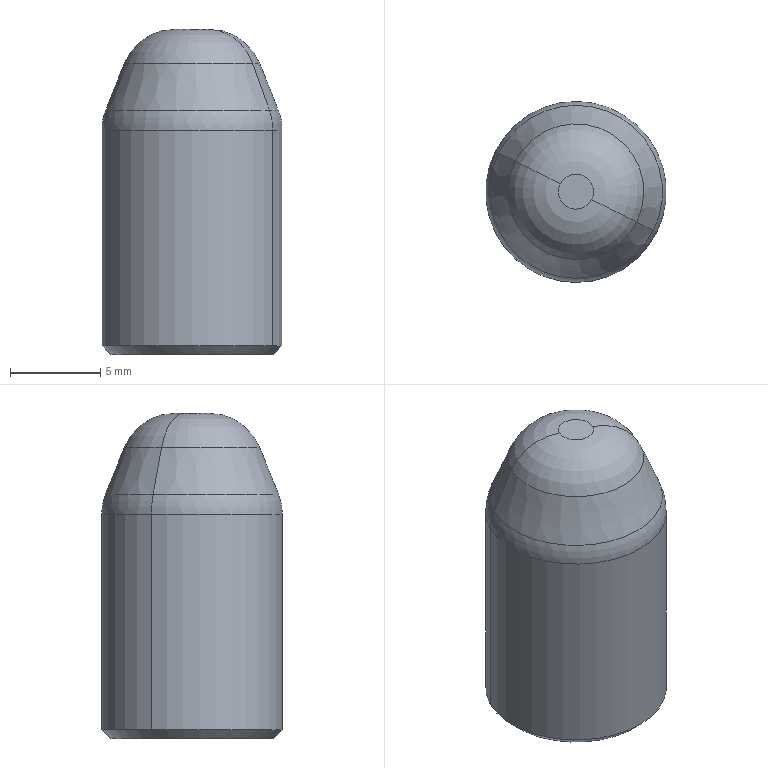Component | SolidWorks | A-C17GuidePin-2 | 1 solid | 16 faces | box 10 x 10 x 18 mm | volume 1171 mm3 | cone 6 | torus 4 | cylinder 4 | plane 2 | commonest cylinder face diameters 3.3 x2 10 x2
build123d program:
from build123d import *

# Parameters (mm, degrees)
SKETCH1_R             = 5
BOSS_EXTRUDE1_DEPTH   = 18
CHAMFER1_SIZE         = 5
CHAMFER1_SIZE2        = 2
M4_TAPPED_HOLE1_D     = 3.3
M4_TAPPED_HOLE1_DEPTH = 10.1
M4_TAPPED_HOLE1_TIP   = 0.9914
CHAMFER2_SIZE         = 0.5
FILLET1_R             = 3


with BuildPart() as part:
    # Sketch1 → Boss-Extrude1 (new body)
    with BuildSketch(Plane.XY):
        Circle(SKETCH1_R)
    extrude(amount=BOSS_EXTRUDE1_DEPTH)

    # Chamfer1
    chamfer1_edges = [part.edges().sort_by_distance(p)[0] for p in [
        (-5, 0, 18),
    ]]
    chamfer1_side = [part.faces().sort_by_distance(p)[0] for p in [
        (-5, 0, 9),
    ]]
    chamfer(chamfer1_edges, length=CHAMFER1_SIZE, length2=CHAMFER1_SIZE2, reference=chamfer1_side[0])

    # M4 Tapped Hole1
    with Locations(Plane(origin=(0, 0, 0), x_dir=(-1, 0, 0), z_dir=(0, 0, -1))):
        with Locations((0, 0)):
            Hole(M4_TAPPED_HOLE1_D / 2, depth=M4_TAPPED_HOLE1_DEPTH)
            with Locations((0, 0, -(M4_TAPPED_HOLE1_DEPTH + M4_TAPPED_HOLE1_TIP / 2))):  # 118° drill point
                Cone(0, M4_TAPPED_HOLE1_D / 2, M4_TAPPED_HOLE1_TIP, mode=Mode.SUBTRACT)

    # Chamfer2
    chamfer2_edges = [part.edges().sort_by_distance(p)[0] for p in [
        (-5, 0, 0),
    ]]
    chamfer(chamfer2_edges, length=CHAMFER2_SIZE)

    # Fillet1
    fillet1_edges = [part.edges().sort_by_distance(p)[0] for p in [
        (-3, 0, 18),
        (-5, 0, 13),
    ]]
    fillet(fillet1_edges, radius=FILLET1_R)


solid = part.part

# Placed as in the assembly
solid = solid.moved(Location((-13.181, 72.568, 23), (0, 0, 0)))
STEP:
#1=COLOUR_RGB('',0.7922,0.8196,0.9333);
#2=FILL_AREA_STYLE_COLOUR('',#1);
#3=FILL_AREA_STYLE('',(#2));
#4=SURFACE_STYLE_FILL_AREA(#3);
#5=SURFACE_SIDE_STYLE('',(#4));
#6=SURFACE_STYLE_USAGE(.BOTH.,#5);
#7=PRESENTATION_STYLE_ASSIGNMENT((#6));
#8=CARTESIAN_POINT('',(-0.3868,2.791,1.54));
#9=VERTEX_POINT('',#8);
#10=CARTESIAN_POINT('',(-0.651,2.923,1.54));
#11=VERTEX_POINT('',#10);
#12=CARTESIAN_POINT('',(-0.5189,2.857,1.54));
#13=DIRECTION('',(0.,0.,-1.));
#14=DIRECTION('',(-0.8939,0.4484,0.));
#15=AXIS2_PLACEMENT_3D('',#12,#13,#14);
#16=CIRCLE('',#15,0.1478);
#17=EDGE_CURVE('',#9,#11,#16,.T.);
#18=ORIENTED_EDGE('',*,*,#17,.F.);
#19=CARTESIAN_POINT('',(-0.4848,2.84,1.614));
#20=VERTEX_POINT('',#19);
#21=CARTESIAN_POINT('',(-0.4848,2.84,1.496));
#22=DIRECTION('',(-0.4484,-0.8939,0.));
#23=DIRECTION('',(0.8939,-0.4484,0.));
#24=AXIS2_PLACEMENT_3D('',#21,#22,#23);
#25=CIRCLE('',#24,0.1181);
#26=EDGE_CURVE('',#9,#20,#25,.T.);
#27=ORIENTED_EDGE('',*,*,#26,.T.);
#28=CARTESIAN_POINT('',(-0.553,2.874,1.614));
#29=VERTEX_POINT('',#28);
#30=CARTESIAN_POINT('',(-0.5189,2.857,1.614));
#31=DIRECTION('',(0.,0.,1.));
#32=DIRECTION('',(-0.8939,0.4484,0.));
#33=AXIS2_PLACEMENT_3D('',#30,#31,#32);
#34=CIRCLE('',#33,0.03815);
#35=EDGE_CURVE('',#29,#20,#34,.T.);
#36=ORIENTED_EDGE('',*,*,#35,.F.);
#37=CARTESIAN_POINT('',(-0.553,2.874,1.496));
#38=DIRECTION('',(0.4484,0.8939,0.));
#39=DIRECTION('',(-0.8939,0.4484,0.));
#40=AXIS2_PLACEMENT_3D('',#37,#38,#39);
#41=CIRCLE('',#40,0.1181);
#42=EDGE_CURVE('',#11,#29,#41,.T.);
#43=ORIENTED_EDGE('',*,*,#42,.F.);
#44=EDGE_LOOP('',(#18,#27,#36,#43));
#45=FACE_OUTER_BOUND('',#44,.T.);
#46=CARTESIAN_POINT('',(-0.5189,2.857,1.496));
#47=DIRECTION('',(0.,0.,1.));
#48=DIRECTION('',(-0.8939,0.4484,0.));
#49=AXIS2_PLACEMENT_3D('',#46,#47,#48);
#50=TOROIDAL_SURFACE('',#49,0.03815,0.1181);
#51=ADVANCED_FACE('',(#45),#50,.T.);
#52=CARTESIAN_POINT('',(-0.343,2.769,1.395));
#53=VERTEX_POINT('',#52);
#54=CARTESIAN_POINT('',(-0.6949,2.945,1.395));
#55=VERTEX_POINT('',#54);
#56=CARTESIAN_POINT('',(-0.5189,2.857,1.395));
#57=DIRECTION('',(0.,0.,-1.));
#58=DIRECTION('',(-0.8939,0.4484,0.));
#59=AXIS2_PLACEMENT_3D('',#56,#57,#58);
#60=CIRCLE('',#59,0.1969);
#61=EDGE_CURVE('',#53,#55,#60,.T.);
#62=ORIENTED_EDGE('',*,*,#61,.F.);
#63=CARTESIAN_POINT('',(-0.3505,2.773,1.438));
#64=VERTEX_POINT('',#63);
#65=CARTESIAN_POINT('',(-0.4485,2.822,1.395));
#66=DIRECTION('',(-0.4484,-0.8939,0.));
#67=DIRECTION('',(0.8939,-0.4484,0.));
#68=AXIS2_PLACEMENT_3D('',#65,#66,#67);
#69=CIRCLE('',#68,0.1181);
#70=EDGE_CURVE('',#53,#64,#69,.T.);
#71=ORIENTED_EDGE('',*,*,#70,.T.);
#72=CARTESIAN_POINT('',(-0.6873,2.941,1.438));
#73=VERTEX_POINT('',#72);
#74=CARTESIAN_POINT('',(-0.5189,2.857,1.438));
#75=DIRECTION('',(0.,0.,1.));
#76=DIRECTION('',(0.8939,-0.4484,0.));
#77=AXIS2_PLACEMENT_3D('',#74,#75,#76);
#78=CIRCLE('',#77,0.1884);
#79=EDGE_CURVE('',#73,#64,#78,.T.);
#80=ORIENTED_EDGE('',*,*,#79,.F.);
#81=CARTESIAN_POINT('',(-0.5893,2.892,1.395));
#82=DIRECTION('',(0.4484,0.8939,0.));
#83=DIRECTION('',(-0.8939,0.4484,0.));
#84=AXIS2_PLACEMENT_3D('',#81,#82,#83);
#85=CIRCLE('',#84,0.1181);
#86=EDGE_CURVE('',#55,#73,#85,.T.);
#87=ORIENTED_EDGE('',*,*,#86,.F.);
#88=EDGE_LOOP('',(#62,#71,#80,#87));
#89=FACE_OUTER_BOUND('',#88,.T.);
#90=CARTESIAN_POINT('',(-0.5189,2.857,1.395));
#91=DIRECTION('',(0.,0.,1.));
#92=DIRECTION('',(-0.8939,0.4484,0.));
#93=AXIS2_PLACEMENT_3D('',#90,#91,#92);
#94=TOROIDAL_SURFACE('',#93,0.07874,0.1181);
#95=ADVANCED_FACE('',(#89),#94,.T.);
#96=CARTESIAN_POINT('',(-0.3606,2.778,0.9055));
#97=VERTEX_POINT('',#96);
#98=CARTESIAN_POINT('',(-0.6773,2.936,0.9055));
#99=VERTEX_POINT('',#98);
#100=CARTESIAN_POINT('',(-0.5189,2.857,0.9055));
#101=DIRECTION('',(0.,0.,-1.));
#102=DIRECTION('',(-0.8939,0.4484,0.));
#103=AXIS2_PLACEMENT_3D('',#100,#101,#102);
#104=CIRCLE('',#103,0.1772);
#105=EDGE_CURVE('',#97,#99,#104,.T.);
#106=ORIENTED_EDGE('',*,*,#105,.F.);
#107=CARTESIAN_POINT('',(-0.343,2.769,0.9252));
#108=VERTEX_POINT('',#107);
#109=CARTESIAN_POINT('',(-0.343,2.769,0.9252));
#110=DIRECTION('',(0.632,-0.317,0.7071));
#111=VECTOR('',#110,39.37);
#112=LINE('',#109,#111);
#113=EDGE_CURVE('',#97,#108,#112,.T.);
#114=ORIENTED_EDGE('',*,*,#113,.T.);
#115=CARTESIAN_POINT('',(-0.6949,2.945,0.9252));
#116=VERTEX_POINT('',#115);
#117=CARTESIAN_POINT('',(-0.5189,2.857,0.9252));
#118=DIRECTION('',(0.,0.,1.));
#119=DIRECTION('',(-0.8939,0.4484,0.));
#120=AXIS2_PLACEMENT_3D('',#117,#118,#119);
#121=CIRCLE('',#120,0.1969);
#122=EDGE_CURVE('',#116,#108,#121,.T.);
#123=ORIENTED_EDGE('',*,*,#122,.F.);
#124=CARTESIAN_POINT('',(-0.6949,2.945,0.9252));
#125=DIRECTION('',(-0.632,0.317,0.7071));
#126=VECTOR('',#125,39.37);
#127=LINE('',#124,#126);
#128=EDGE_CURVE('',#99,#116,#127,.T.);
#129=ORIENTED_EDGE('',*,*,#128,.F.);
#130=EDGE_LOOP('',(#106,#114,#123,#129));
#131=FACE_OUTER_BOUND('',#130,.T.);
#132=CARTESIAN_POINT('',(-0.5189,2.857,0.9252));
#133=DIRECTION('',(0.,0.,1.));
#134=DIRECTION('',(-0.8939,0.4484,0.));
#135=AXIS2_PLACEMENT_3D('',#132,#133,#134);
#136=CONICAL_SURFACE('',#135,0.1969,0.7854);
#137=ADVANCED_FACE('',(#131),#136,.T.);
#138=CARTESIAN_POINT('',(-0.577,2.886,1.303));
#139=VERTEX_POINT('',#138);
#140=CARTESIAN_POINT('',(-0.4609,2.828,1.303));
#141=VERTEX_POINT('',#140);
#142=CARTESIAN_POINT('',(-0.5189,2.857,1.303));
#143=DIRECTION('',(0.,0.,-1.));
#144=DIRECTION('',(0.8939,-0.4484,0.));
#145=AXIS2_PLACEMENT_3D('',#142,#143,#144);
#146=CIRCLE('',#145,0.06496);
#147=EDGE_CURVE('',#139,#141,#146,.T.);
#148=ORIENTED_EDGE('',*,*,#147,.F.);
#149=CARTESIAN_POINT('',(-0.577,2.886,0.9055));
#150=VERTEX_POINT('',#149);
#151=CARTESIAN_POINT('',(-0.577,2.886,0.9055));
#152=DIRECTION('',(0.,0.,-1.));
#153=VECTOR('',#152,39.37);
#154=LINE('',#151,#153);
#155=EDGE_CURVE('',#139,#150,#154,.T.);
#156=ORIENTED_EDGE('',*,*,#155,.T.);
#157=CARTESIAN_POINT('',(-0.4609,2.828,0.9055));
#158=VERTEX_POINT('',#157);
#159=CARTESIAN_POINT('',(-0.5189,2.857,0.9055));
#160=DIRECTION('',(0.,0.,-1.));
#161=DIRECTION('',(0.8939,-0.4484,0.));
#162=AXIS2_PLACEMENT_3D('',#159,#160,#161);
#163=CIRCLE('',#162,0.06496);
#164=EDGE_CURVE('',#150,#158,#163,.T.);
#165=ORIENTED_EDGE('',*,*,#164,.T.);
#166=CARTESIAN_POINT('',(-0.4609,2.828,0.9055));
#167=DIRECTION('',(0.,0.,-1.));
#168=VECTOR('',#167,39.37);
#169=LINE('',#166,#168);
#170=EDGE_CURVE('',#141,#158,#169,.T.);
#171=ORIENTED_EDGE('',*,*,#170,.F.);
#172=EDGE_LOOP('',(#148,#156,#165,#171));
#173=FACE_OUTER_BOUND('',#172,.T.);
#174=CARTESIAN_POINT('',(-0.5189,2.857,0.9055));
#175=DIRECTION('',(0.,0.,-1.));
#176=DIRECTION('',(0.8939,-0.4484,0.));
#177=AXIS2_PLACEMENT_3D('',#174,#175,#176);
#178=CYLINDRICAL_SURFACE('',#177,0.06496);
#179=ADVANCED_FACE('',(#173),#178,.F.);
#180=CARTESIAN_POINT('',(-0.5189,2.857,1.342));
#181=VERTEX_POINT('',#180);
#182=CARTESIAN_POINT('',(-0.4609,2.828,1.303));
#183=DIRECTION('',(0.7662,-0.3843,-0.515));
#184=VECTOR('',#183,39.37);
#185=LINE('',#182,#184);
#186=EDGE_CURVE('',#181,#141,#185,.T.);
#187=ORIENTED_EDGE('',*,*,#186,.F.);
#188=CARTESIAN_POINT('',(-0.577,2.886,1.303));
#189=DIRECTION('',(-0.7662,0.3843,-0.515));
#190=VECTOR('',#189,39.37);
#191=LINE('',#188,#190);
#192=EDGE_CURVE('',#181,#139,#191,.T.);
#193=ORIENTED_EDGE('',*,*,#192,.T.);
#194=ORIENTED_EDGE('',*,*,#147,.T.);
#195=EDGE_LOOP('',(#187,#193,#194));
#196=FACE_OUTER_BOUND('',#195,.T.);
#197=CARTESIAN_POINT('',(-0.5189,2.857,1.303));
#198=DIRECTION('',(0.,0.,-1.));
#199=DIRECTION('',(0.8939,-0.4484,0.));
#200=AXIS2_PLACEMENT_3D('',#197,#198,#199);
#201=CONICAL_SURFACE('',#200,0.06496,1.03);
#202=ADVANCED_FACE('',(#196),#201,.F.);
#203=ORIENTED_EDGE('',*,*,#17,.T.);
#204=CARTESIAN_POINT('',(-0.6245,2.91,1.614));
#205=DIRECTION('',(-0.332,0.1665,-0.9285));
#206=VECTOR('',#205,39.37);
#207=LINE('',#204,#206);
#208=EDGE_CURVE('',#11,#73,#207,.T.);
#209=ORIENTED_EDGE('',*,*,#208,.T.);
#210=ORIENTED_EDGE('',*,*,#79,.T.);
#211=CARTESIAN_POINT('',(-0.4134,2.804,1.614));
#212=DIRECTION('',(0.332,-0.1665,-0.9285));
#213=VECTOR('',#212,39.37);
#214=LINE('',#211,#213);
#215=EDGE_CURVE('',#9,#64,#214,.T.);
#216=ORIENTED_EDGE('',*,*,#215,.F.);
#217=EDGE_LOOP('',(#203,#209,#210,#216));
#218=FACE_OUTER_BOUND('',#217,.T.);
#219=CARTESIAN_POINT('',(-0.5189,2.857,1.614));
#220=DIRECTION('',(0.,0.,-1.));
#221=DIRECTION('',(0.8939,-0.4484,0.));
#222=AXIS2_PLACEMENT_3D('',#219,#220,#221);
#223=CONICAL_SURFACE('',#222,0.1181,0.3805);
#224=ADVANCED_FACE('',(#218),#223,.T.);
#225=ORIENTED_EDGE('',*,*,#61,.T.);
#226=CARTESIAN_POINT('',(-0.6949,2.945,1.614));
#227=DIRECTION('',(0.,0.,-1.));
#228=VECTOR('',#227,39.37);
#229=LINE('',#226,#228);
#230=EDGE_CURVE('',#55,#116,#229,.T.);
#231=ORIENTED_EDGE('',*,*,#230,.T.);
#232=ORIENTED_EDGE('',*,*,#122,.T.);
#233=CARTESIAN_POINT('',(-0.343,2.769,1.614));
#234=DIRECTION('',(0.,0.,-1.));
#235=VECTOR('',#234,39.37);
#236=LINE('',#233,#235);
#237=EDGE_CURVE('',#53,#108,#236,.T.);
#238=ORIENTED_EDGE('',*,*,#237,.F.);
#239=EDGE_LOOP('',(#225,#231,#232,#238));
#240=FACE_OUTER_BOUND('',#239,.T.);
#241=CARTESIAN_POINT('',(-0.5189,2.857,1.614));
#242=DIRECTION('',(0.,0.,-1.));
#243=DIRECTION('',(0.8939,-0.4484,0.));
#244=AXIS2_PLACEMENT_3D('',#241,#242,#243);
#245=CYLINDRICAL_SURFACE('',#244,0.1969);
#246=ADVANCED_FACE('',(#240),#245,.T.);
#247=ORIENTED_EDGE('',*,*,#230,.F.);
#248=CARTESIAN_POINT('',(-0.5189,2.857,1.395));
#249=DIRECTION('',(0.,0.,-1.));
#250=DIRECTION('',(-0.8939,0.4484,0.));
#251=AXIS2_PLACEMENT_3D('',#248,#249,#250);
#252=CIRCLE('',#251,0.1969);
#253=EDGE_CURVE('',#55,#53,#252,.T.);
#254=ORIENTED_EDGE('',*,*,#253,.T.);
#255=ORIENTED_EDGE('',*,*,#237,.T.);
#256=CARTESIAN_POINT('',(-0.5189,2.857,0.9252));
#257=DIRECTION('',(0.,0.,1.));
#258=DIRECTION('',(-0.8939,0.4484,0.));
#259=AXIS2_PLACEMENT_3D('',#256,#257,#258);
#260=CIRCLE('',#259,0.1969);
#261=EDGE_CURVE('',#108,#116,#260,.T.);
#262=ORIENTED_EDGE('',*,*,#261,.T.);
#263=EDGE_LOOP('',(#247,#254,#255,#262));
#264=FACE_OUTER_BOUND('',#263,.T.);
#265=CARTESIAN_POINT('',(-0.5189,2.857,1.614));
#266=DIRECTION('',(0.,0.,-1.));
#267=DIRECTION('',(0.8939,-0.4484,0.));
#268=AXIS2_PLACEMENT_3D('',#265,#266,#267);
#269=CYLINDRICAL_SURFACE('',#268,0.1969);
#270=ADVANCED_FACE('',(#264),#269,.T.);
#271=ORIENTED_EDGE('',*,*,#35,.T.);
#272=CARTESIAN_POINT('',(-0.5189,2.857,1.614));
#273=DIRECTION('',(0.,0.,1.));
#274=DIRECTION('',(-0.8939,0.4484,0.));
#275=AXIS2_PLACEMENT_3D('',#272,#273,#274);
#276=CIRCLE('',#275,0.03815);
#277=EDGE_CURVE('',#20,#29,#276,.T.);
#278=ORIENTED_EDGE('',*,*,#277,.T.);
#279=EDGE_LOOP('',(#271,#278));
#280=FACE_OUTER_BOUND('',#279,.T.);
#281=CARTESIAN_POINT('',(-0.5189,2.857,1.614));
#282=DIRECTION('',(0.,0.,1.));
#283=DIRECTION('',(-0.8939,0.4484,0.));
#284=AXIS2_PLACEMENT_3D('',#281,#282,#283);
#285=PLANE('',#284);
#286=ADVANCED_FACE('',(#280),#285,.T.);
#287=CARTESIAN_POINT('',(-0.5189,2.857,0.9055));
#288=DIRECTION('',(0.,0.,-1.));
#289=DIRECTION('',(-0.8939,0.4484,0.));
#290=AXIS2_PLACEMENT_3D('',#287,#288,#289);
#291=CIRCLE('',#290,0.1772);
#292=EDGE_CURVE('',#99,#97,#291,.T.);
#293=ORIENTED_EDGE('',*,*,#292,.T.);
#294=ORIENTED_EDGE('',*,*,#105,.T.);
#295=EDGE_LOOP('',(#293,#294));
#296=FACE_OUTER_BOUND('',#295,.T.);
#297=CARTESIAN_POINT('',(-0.5189,2.857,0.9055));
#298=DIRECTION('',(0.,0.,-1.));
#299=DIRECTION('',(0.8939,-0.4484,0.));
#300=AXIS2_PLACEMENT_3D('',#297,#298,#299);
#301=CIRCLE('',#300,0.06496);
#302=EDGE_CURVE('',#158,#150,#301,.T.);
#303=ORIENTED_EDGE('',*,*,#302,.F.);
#304=ORIENTED_EDGE('',*,*,#164,.F.);
#305=EDGE_LOOP('',(#303,#304));
#306=FACE_BOUND('',#305,.T.);
#307=CARTESIAN_POINT('',(-0.5189,2.857,0.9055));
#308=DIRECTION('',(0.,0.,1.));
#309=DIRECTION('',(-0.8939,0.4484,0.));
#310=AXIS2_PLACEMENT_3D('',#307,#308,#309);
#311=PLANE('',#310);
#312=ADVANCED_FACE('',(#296,#306),#311,.F.);
#313=ORIENTED_EDGE('',*,*,#208,.F.);
#314=CARTESIAN_POINT('',(-0.5189,2.857,1.54));
#315=DIRECTION('',(0.,0.,-1.));
#316=DIRECTION('',(-0.8939,0.4484,0.));
#317=AXIS2_PLACEMENT_3D('',#314,#315,#316);
#318=CIRCLE('',#317,0.1478);
#319=EDGE_CURVE('',#11,#9,#318,.T.);
#320=ORIENTED_EDGE('',*,*,#319,.T.);
#321=ORIENTED_EDGE('',*,*,#215,.T.);
#322=CARTESIAN_POINT('',(-0.5189,2.857,1.438));
#323=DIRECTION('',(0.,0.,1.));
#324=DIRECTION('',(0.8939,-0.4484,0.));
#325=AXIS2_PLACEMENT_3D('',#322,#323,#324);
#326=CIRCLE('',#325,0.1884);
#327=EDGE_CURVE('',#64,#73,#326,.T.);
#328=ORIENTED_EDGE('',*,*,#327,.T.);
#329=EDGE_LOOP('',(#313,#320,#321,#328));
#330=FACE_OUTER_BOUND('',#329,.T.);
#331=CARTESIAN_POINT('',(-0.5189,2.857,1.614));
#332=DIRECTION('',(0.,0.,-1.));
#333=DIRECTION('',(0.8939,-0.4484,0.));
#334=AXIS2_PLACEMENT_3D('',#331,#332,#333);
#335=CONICAL_SURFACE('',#334,0.1181,0.3805);
#336=ADVANCED_FACE('',(#330),#335,.T.);
#337=ORIENTED_EDGE('',*,*,#192,.F.);
#338=ORIENTED_EDGE('',*,*,#186,.T.);
#339=CARTESIAN_POINT('',(-0.5189,2.857,1.303));
#340=DIRECTION('',(0.,0.,-1.));
#341=DIRECTION('',(0.8939,-0.4484,0.));
#342=AXIS2_PLACEMENT_3D('',#339,#340,#341);
#343=CIRCLE('',#342,0.06496);
#344=EDGE_CURVE('',#141,#139,#343,.T.);
#345=ORIENTED_EDGE('',*,*,#344,.T.);
#346=EDGE_LOOP('',(#337,#338,#345));
#347=FACE_OUTER_BOUND('',#346,.T.);
#348=CARTESIAN_POINT('',(-0.5189,2.857,1.303));
#349=DIRECTION('',(0.,0.,-1.));
#350=DIRECTION('',(0.8939,-0.4484,0.));
#351=AXIS2_PLACEMENT_3D('',#348,#349,#350);
#352=CONICAL_SURFACE('',#351,0.06496,1.03);
#353=ADVANCED_FACE('',(#347),#352,.F.);
#354=ORIENTED_EDGE('',*,*,#155,.F.);
#355=ORIENTED_EDGE('',*,*,#344,.F.);
#356=ORIENTED_EDGE('',*,*,#170,.T.);
#357=ORIENTED_EDGE('',*,*,#302,.T.);
#358=EDGE_LOOP('',(#354,#355,#356,#357));
#359=FACE_OUTER_BOUND('',#358,.T.);
#360=CARTESIAN_POINT('',(-0.5189,2.857,0.9055));
#361=DIRECTION('',(0.,0.,-1.));
#362=DIRECTION('',(0.8939,-0.4484,0.));
#363=AXIS2_PLACEMENT_3D('',#360,#361,#362);
#364=CYLINDRICAL_SURFACE('',#363,0.06496);
#365=ADVANCED_FACE('',(#359),#364,.F.);
#366=ORIENTED_EDGE('',*,*,#113,.F.);
#367=ORIENTED_EDGE('',*,*,#292,.F.);
#368=ORIENTED_EDGE('',*,*,#128,.T.);
#369=ORIENTED_EDGE('',*,*,#261,.F.);
#370=EDGE_LOOP('',(#366,#367,#368,#369));
#371=FACE_OUTER_BOUND('',#370,.T.);
#372=CARTESIAN_POINT('',(-0.5189,2.857,0.9252));
#373=DIRECTION('',(0.,0.,1.));
#374=DIRECTION('',(-0.8939,0.4484,0.));
#375=AXIS2_PLACEMENT_3D('',#372,#373,#374);
#376=CONICAL_SURFACE('',#375,0.1969,0.7854);
#377=ADVANCED_FACE('',(#371),#376,.T.);
#378=ORIENTED_EDGE('',*,*,#70,.F.);
#379=ORIENTED_EDGE('',*,*,#253,.F.);
#380=ORIENTED_EDGE('',*,*,#86,.T.);
#381=ORIENTED_EDGE('',*,*,#327,.F.);
#382=EDGE_LOOP('',(#378,#379,#380,#381));
#383=FACE_OUTER_BOUND('',#382,.T.);
#384=CARTESIAN_POINT('',(-0.5189,2.857,1.395));
#385=DIRECTION('',(0.,0.,1.));
#386=DIRECTION('',(-0.8939,0.4484,0.));
#387=AXIS2_PLACEMENT_3D('',#384,#385,#386);
#388=TOROIDAL_SURFACE('',#387,0.07874,0.1181);
#389=ADVANCED_FACE('',(#383),#388,.T.);
#390=ORIENTED_EDGE('',*,*,#26,.F.);
#391=ORIENTED_EDGE('',*,*,#319,.F.);
#392=ORIENTED_EDGE('',*,*,#42,.T.);
#393=ORIENTED_EDGE('',*,*,#277,.F.);
#394=EDGE_LOOP('',(#390,#391,#392,#393));
#395=FACE_OUTER_BOUND('',#394,.T.);
#396=CARTESIAN_POINT('',(-0.5189,2.857,1.496));
#397=DIRECTION('',(0.,0.,1.));
#398=DIRECTION('',(-0.8939,0.4484,0.));
#399=AXIS2_PLACEMENT_3D('',#396,#397,#398);
#400=TOROIDAL_SURFACE('',#399,0.03815,0.1181);
#401=ADVANCED_FACE('',(#395),#400,.T.);
#402=CLOSED_SHELL('',(#51,#95,#137,#179,#202,#224,#246,#270,#286,#312,#336,#353,#365,#377,#389,#401));
#403=MANIFOLD_SOLID_BREP('',#402);
#404=STYLED_ITEM('',(#7),#403);
#405=PRESENTATION_LAYER_ASSIGNMENT('','',(#404));
#406=(LENGTH_UNIT()NAMED_UNIT(*)SI_UNIT($,.METRE.));
#407=LENGTH_MEASURE_WITH_UNIT(LENGTH_MEASURE(0.0254),#406);
#408=DIMENSIONAL_EXPONENTS(1.,0.,0.,0.,0.,0.,0.);
#409=(CONVERSION_BASED_UNIT('',#407)LENGTH_UNIT()NAMED_UNIT(#408));
#410=UNCERTAINTY_MEASURE_WITH_UNIT(LENGTH_MEASURE(0.00001),#409,'','');
#411=(NAMED_UNIT(*)PLANE_ANGLE_UNIT()SI_UNIT($,.RADIAN.));
#412=(NAMED_UNIT(*)SI_UNIT($,.STERADIAN.)SOLID_ANGLE_UNIT());
#413=(GEOMETRIC_REPRESENTATION_CONTEXT(3)GLOBAL_UNCERTAINTY_ASSIGNED_CONTEXT((#410))GLOBAL_UNIT_ASSIGNED_CONTEXT((#409,#411,#412))REPRESENTATION_CONTEXT('',''));
#414=MECHANICAL_DESIGN_GEOMETRIC_PRESENTATION_REPRESENTATION('',(#404),#413);
#415=CARTESIAN_POINT('',(0.,0.,0.));
#416=DIRECTION('',(0.,0.,1.));
#417=DIRECTION('',(1.,0.,0.));
#418=AXIS2_PLACEMENT_3D('',#415,#416,#417);
#419=(LENGTH_UNIT()NAMED_UNIT(*)SI_UNIT($,.METRE.));
#420=LENGTH_MEASURE_WITH_UNIT(LENGTH_MEASURE(0.0254),#419);
#421=DIMENSIONAL_EXPONENTS(1.,0.,0.,0.,0.,0.,0.);
#422=(CONVERSION_BASED_UNIT('',#420)LENGTH_UNIT()NAMED_UNIT(#421));
#423=UNCERTAINTY_MEASURE_WITH_UNIT(LENGTH_MEASURE(0.00001),#422,'','');
#424=(NAMED_UNIT(*)PLANE_ANGLE_UNIT()SI_UNIT($,.RADIAN.));
#425=(NAMED_UNIT(*)SI_UNIT($,.STERADIAN.)SOLID_ANGLE_UNIT());
#426=(GEOMETRIC_REPRESENTATION_CONTEXT(3)GLOBAL_UNCERTAINTY_ASSIGNED_CONTEXT((#423))GLOBAL_UNIT_ASSIGNED_CONTEXT((#422,#424,#425))REPRESENTATION_CONTEXT('',''));
#427=ADVANCED_BREP_SHAPE_REPRESENTATION('',(#403,#418),#426);